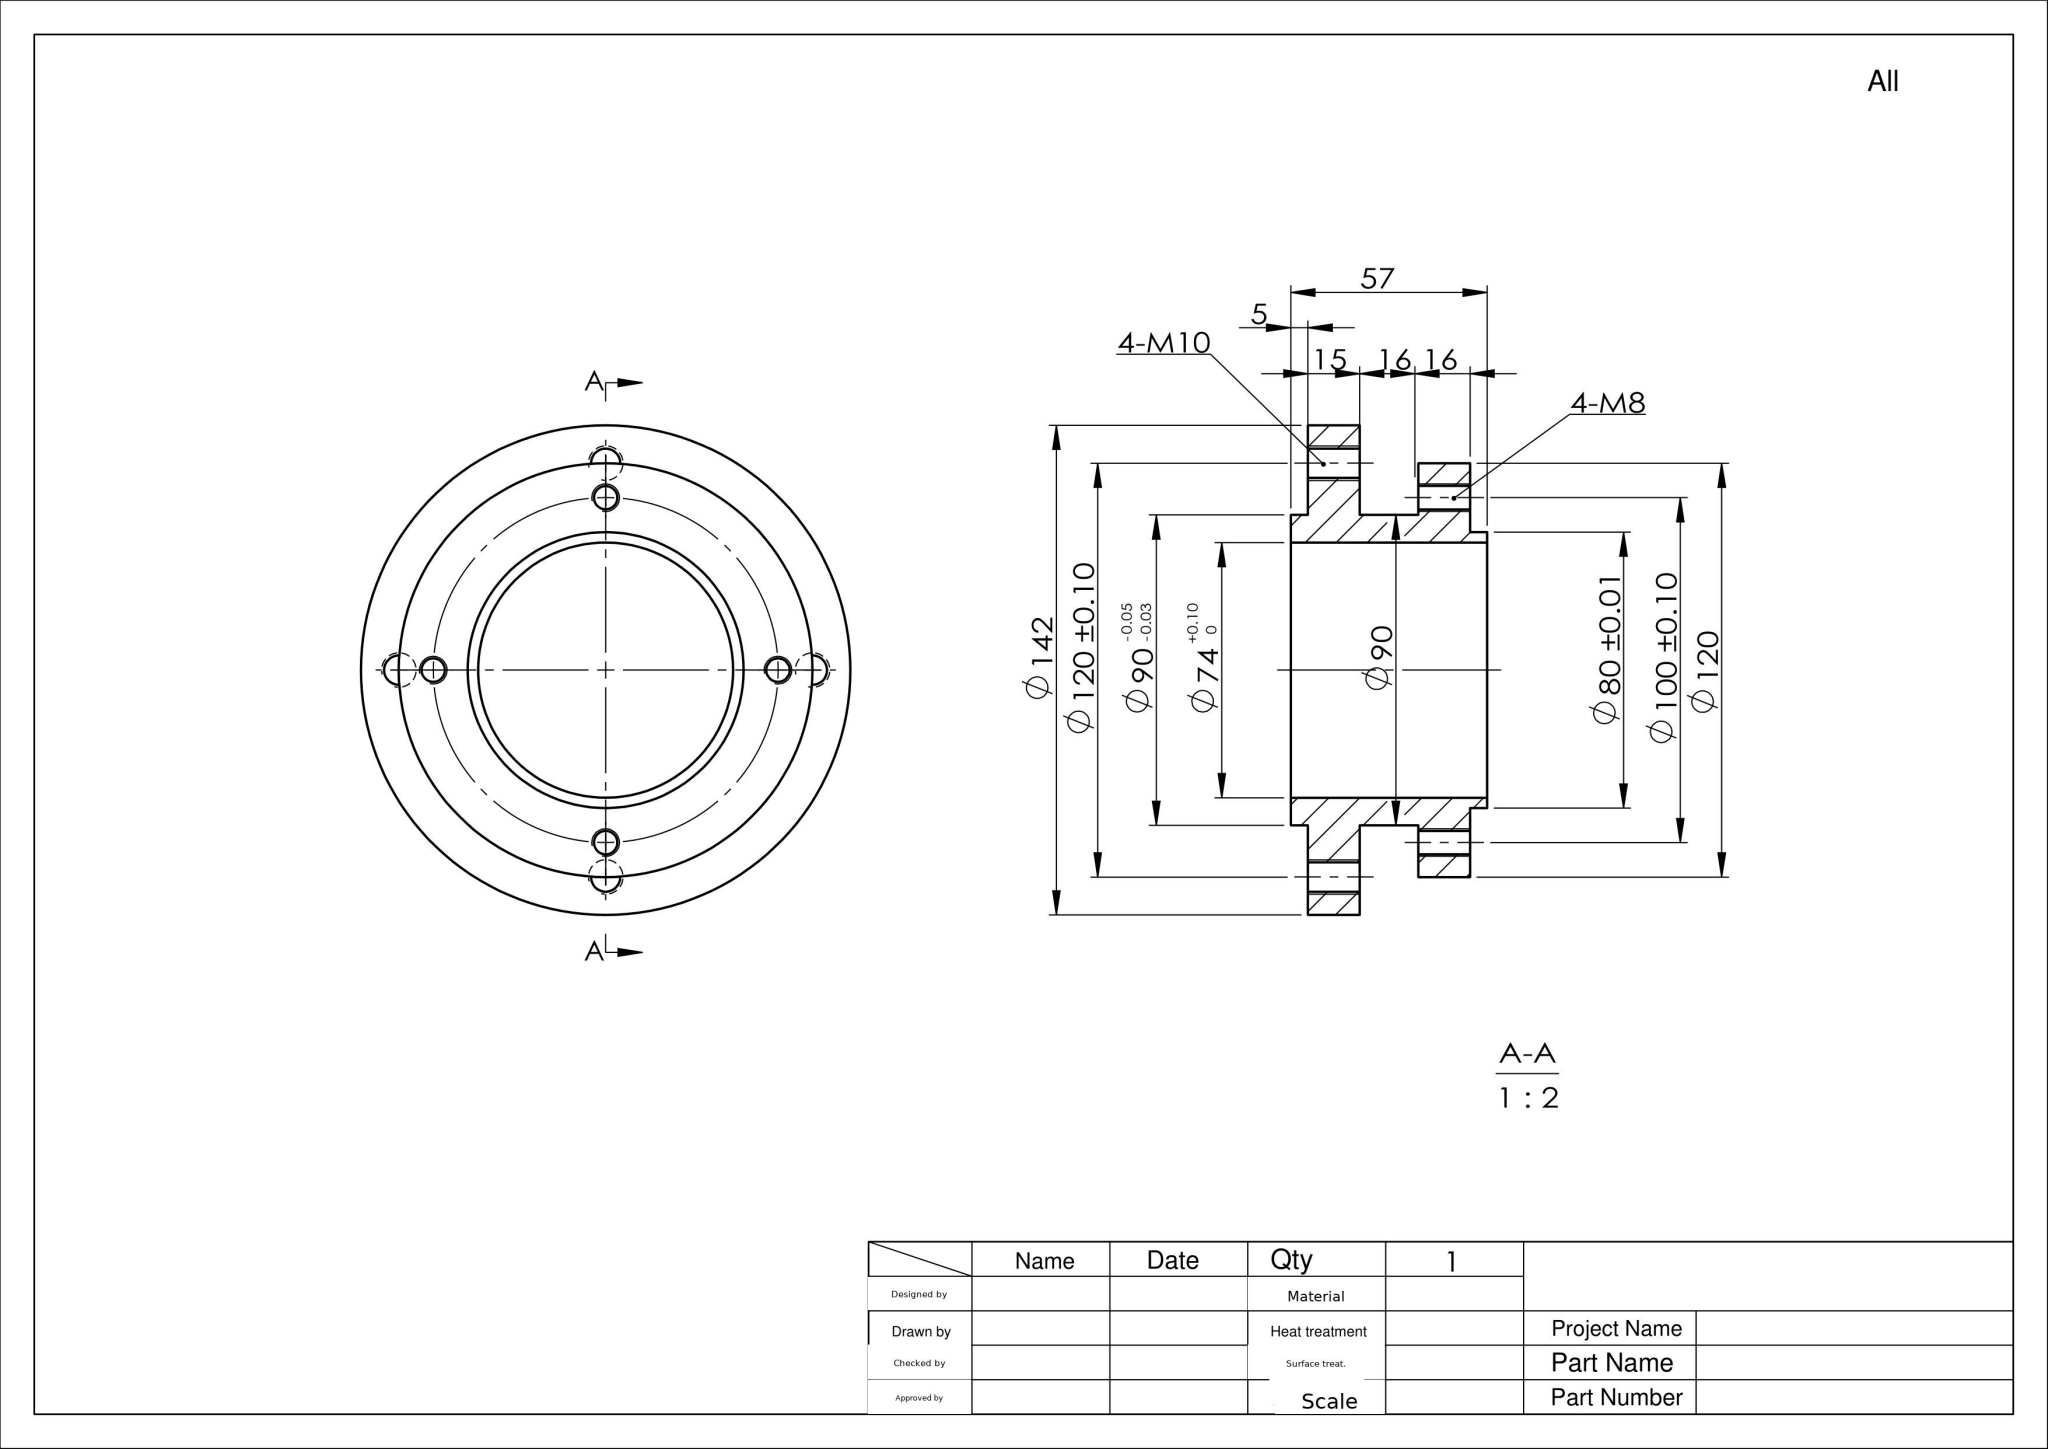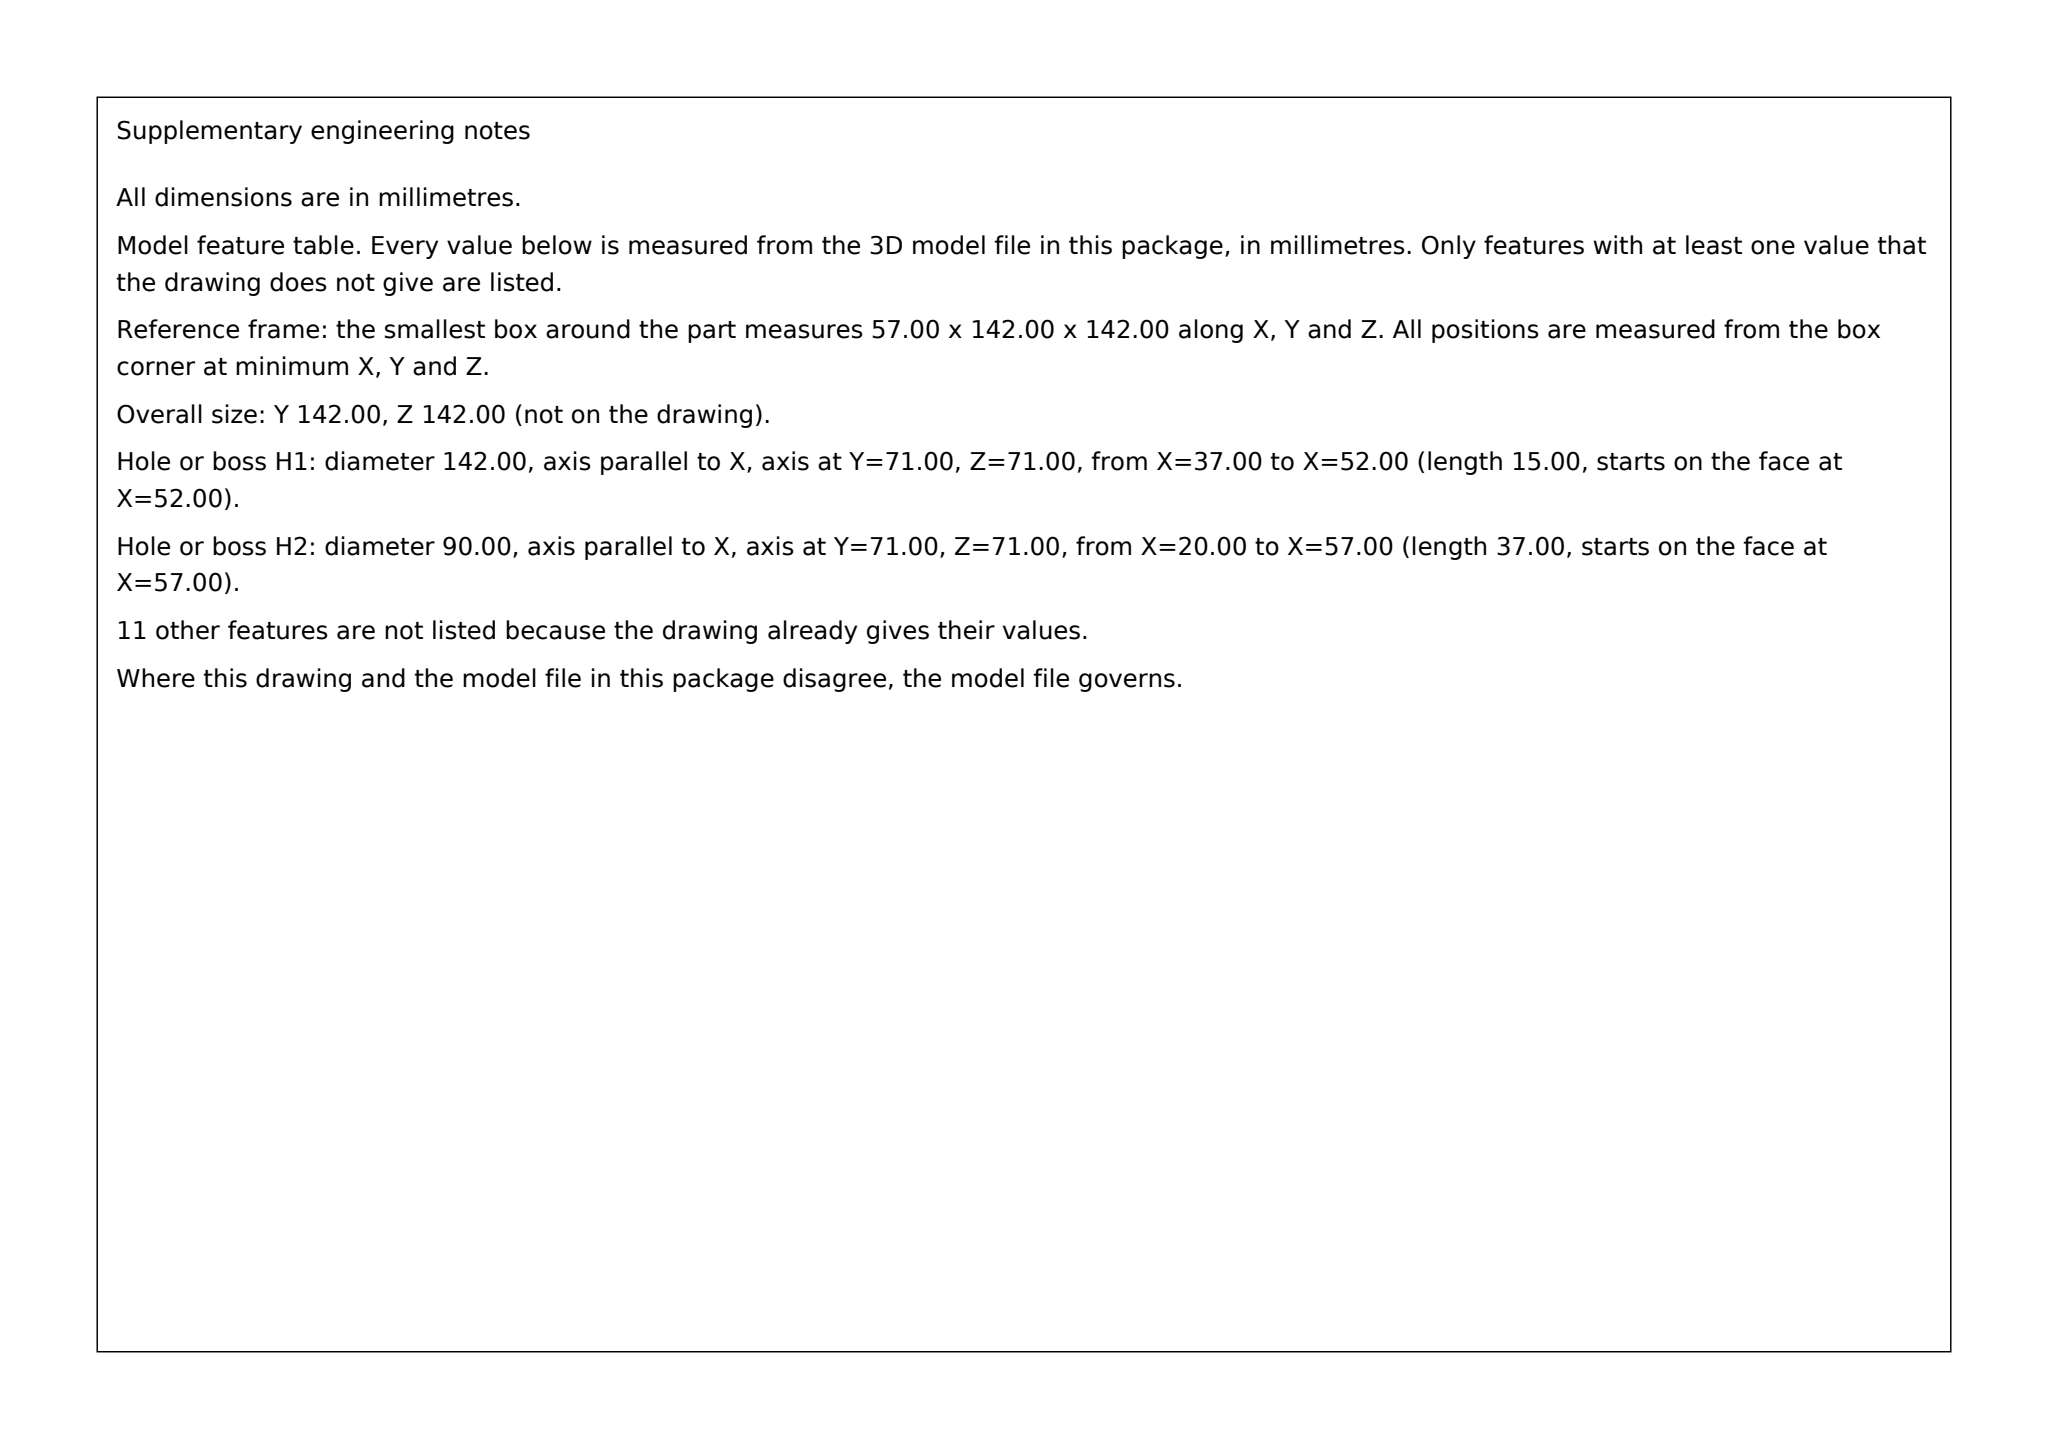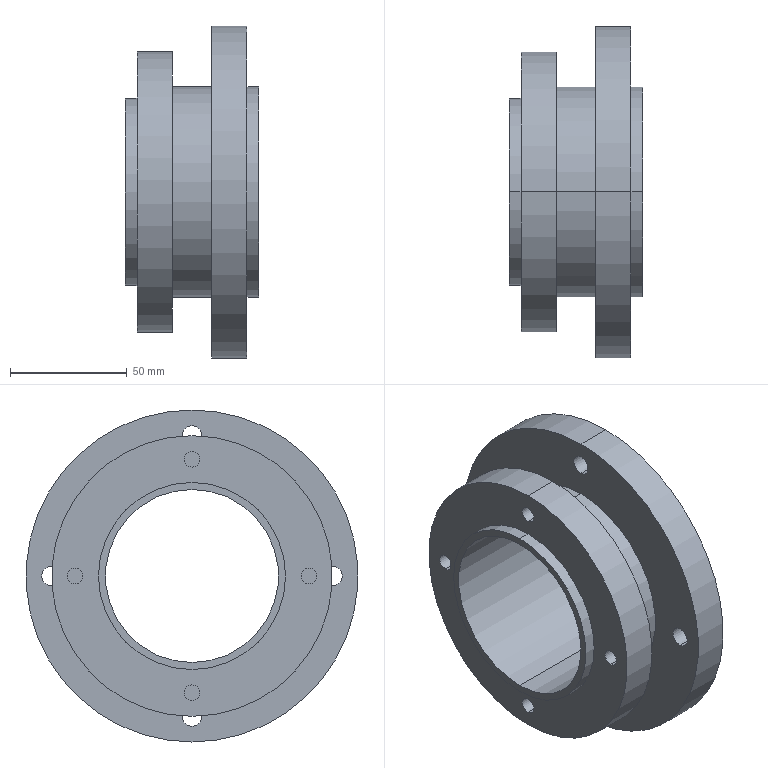Part | SolidWorks | mm | 1 solid | 34 faces | box 57 x 142 x 142 mm | volume 321557 mm3 | cylinder 28 | plane 6 | commonest cylinder face diameters 6.8 x8 8.5 x8 90 x4 80 x2 120 x2 142 x2 74 x2
build123d program:
from build123d import *

# Parameters (mm, degrees)
CIRPATTERN1_COUNT = 4
CIRPATTERN2_COUNT = 4


with BuildPart() as part:
    # Sketch1 → Revolve1 (revolve)
    with BuildSketch(Plane.XY, mode=Mode.PRIVATE) as revolve1_sk:
        Polygon((0, 37), (0, 40), (5, 40), (5, 60), (20, 60), (20, 45), (37, 45), (37, 71), (52, 71), (52, 45), (57, 45), (57, 37), align=None)
    revolve(revolve1_sk.sketch.rotate(Axis((0, 0, 0), (1, 0, 0)), 90), axis=Axis((0, 0, 0), (1, 0, 0)))

    # Sketch3 → M10 Tapped Hole1 (revolve, cut)
    with BuildSketch(Plane(origin=(52, 60, 0), x_dir=(0, 0, -1), z_dir=(0, 1, 0))):
        Polygon((0, 0), (0, 17.554), (4.25, 15), (4.25, 0), align=None)
    m10_tapped_hole1 = revolve(axis=Axis((58.35, 60, 0), (-1, 0, 0)), mode=Mode.SUBTRACT)

    # CirPattern1: M10 Tapped Hole1 ×4 about axis
    cirpattern1_axis = Axis((0, 0, 0), (1, 0, 0))
    for i in range(1, CIRPATTERN1_COUNT):
        add(m10_tapped_hole1.rotate(cirpattern1_axis, i * 360 / CIRPATTERN1_COUNT), mode=Mode.SUBTRACT)

    # Sketch5 → M8 Tapped Hole1 (revolve, cut)
    with BuildSketch(Plane(origin=(5, 50, 0), x_dir=(0, 0, 1), z_dir=(0, 1, 0))):
        Polygon((0, 0), (0, 17.043), (3.4, 15), (3.4, 0), align=None)
    m8_tapped_hole1 = revolve(axis=Axis((-1.35, 50, 0), (1, 0, 0)), mode=Mode.SUBTRACT)

    # CirPattern2: M8 Tapped Hole1 ×4 about axis
    cirpattern2_axis = Axis((0, 0, 0), (1, 0, 0))
    for i in range(1, CIRPATTERN2_COUNT):
        add(m8_tapped_hole1.rotate(cirpattern2_axis, i * 360 / CIRPATTERN2_COUNT), mode=Mode.SUBTRACT)


solid = part.part